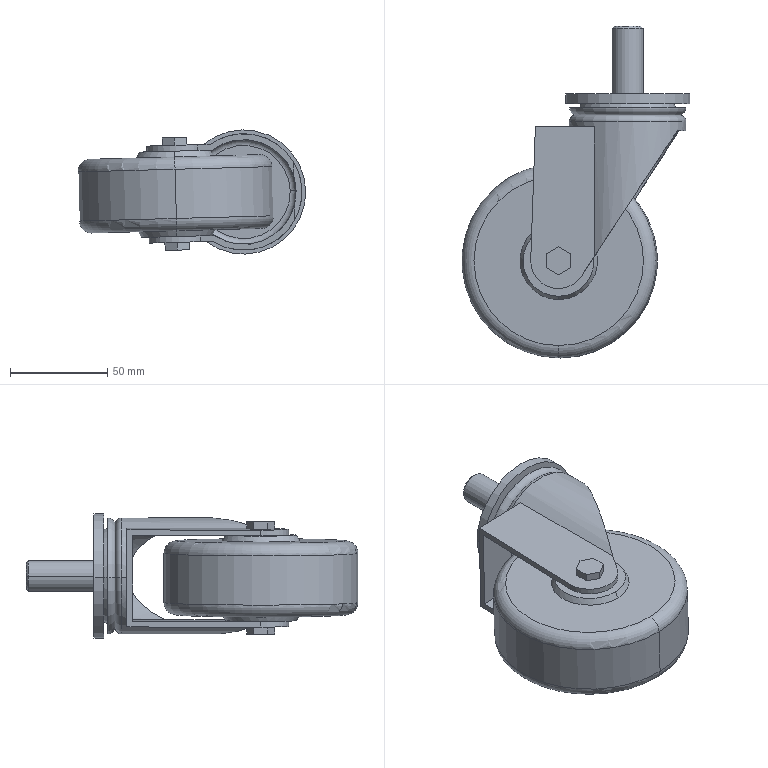Component | SolidWorks | Caster-WHB31-D100-P-3 | 1 solid | 64 faces | volume 376534 mm3 | plane 34 | cylinder 12 | torus 10 | cone 8 | commonest cylinder face diameters 100 x2 54 x2 64 x2 16 x2 60 x2 28.571 x2